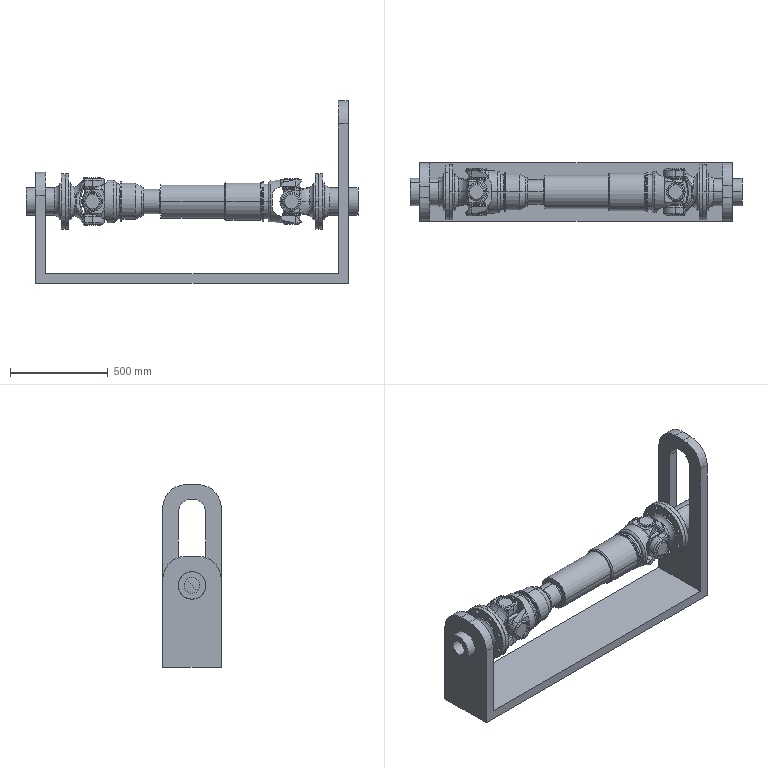Assembly | NX | mm | 10 component files | 38 solids | 702 faces | box 1700 x 300 x 936.56 mm | volume 77228193 mm3 | cylinder 314 | plane 174 | torus 122 | spline 48 | cone 36 | sphere 8 | commonest cylinder face diameters 20.1 x64 14 x56 83 x40 92 x20 90 x16 30 x8 24 x8 157.541 x8
Bill of materials:
unnamed part 1 | 2 |  | Flanged fork: a circular flat flange with a short raised hub, carrying two parallel lugs (a fork shape) that each have a round bore. The two bores share one axis.
unnamed part 2 | 1 |  | Fork attached to a stepped cylindrical shaft: a two-lug fork with coaxial round bores at one end, a larger round body with a raised ring and stepped diameters, and then a long smaller-diameter shaft.
unnamed part 3 | 1 |  | U-shaped bracket made from flat strip: a long flat base with two upright tabs at the ends that have rounded tops. One upright is taller than the other. One tab has a round hole and the other has an elongated slot.
unnamed part 4 | 1 |  | Fork attached to a cylindrical tube or shaft: a two-lug fork with coaxial round bores at one end, a short collar with a ring groove or rib, a larger cylindrical sleeve section, and then a long plain cylinder of smaller diameter.
unnamed part 5 | 1 |  | Plain solid cylinder with flat ends. Its length is about equal to its diameter.
unnamed part 6 | 2 |  | Cross-shaped body with four cylindrical arms (trunnions) sticking out from a rounded square centre block. The arms lie in one plane and are at 90° to each other.
unnamed part 7 | 2 |  | Flanged tube or spigot: a circular flat flange with eight bolt holes, and a cylindrical body sticking out from one side with a curved fillet transition. The flange face has a large central recess shaped like a bowl or counterbore.
Mates:
1. fix | model82 1 component
2. distance | model82 1 face | BRIDA2_587_Predeterminado_Como_mecanizada 1 face
3. touch align | model82 1 face | BRIDA2_587_Predeterminado_Como_mecanizada 1 face
4. touch align | BRIDA2_587_Predeterminado_Como_mecanizada 1 face | BRIDA_587_Predeterminado_Como_mecanizada 1 face
5. touch align | BRIDA_587_Predeterminado_Como_mecanizada 1 face | BRIDA2_587_Predeterminado_Como_mecanizada 1 face
6. touch align | BRIDA2_587_Predeterminado_Como_mecanizada 1 face | BRIDA_587_Predeterminado_Como_mecanizada 1 face
7. touch align | CRUZ_587_Predeterminado_Como_mecanizada 1 face | BRIDA_587_Predeterminado_Como_mecanizada 1 face
8. center | BRIDA_587_Predeterminado_Como_mecanizada 1 face | BRIDA_587_Predeterminado_Como_mecanizada 1 face | CRUZ_587_Predeterminado_Como_mecanizada 1 face | CRUZ_587_Predeterminado_Como_mecanizada 1 face
9. center | BRAZO_Predeterminado_Como_mecanizada 1 face | BRAZO_Predeterminado_Como_mecanizada 1 face | CRUZ_587_Predeterminado_Como_mecanizada 1 face | CRUZ_587_Predeterminado_Como_mecanizada 1 face
10. touch align | BRAZO_Predeterminado_Como_mecanizada 1 face | CRUZ_587_Predeterminado_Como_mecanizada 1 face
11. touch align | BRAZO_HUECO_Predeterminado_Como_mecanizada 1 face | BRAZO_Predeterminado_Como_mecanizada 1 face
12. touch align | CRUZ_587_Predeterminado_Como_mecanizada 2 face | BRAZO_HUECO_Predeterminado_Como_mecanizada 1 face
13. center | BRAZO_HUECO_Predeterminado_Como_mecanizada 1 face | BRAZO_HUECO_Predeterminado_Como_mecanizada 1 face | CRUZ_587_Predeterminado_Como_mecanizada 2 face | CRUZ_587_Predeterminado_Como_mecanizada 2 face
14. touch align | BRIDA_587_Predeterminado_Como_mecanizada 2 face | CRUZ_587_Predeterminado_Como_mecanizada 2 face
15. center | BRIDA_587_Predeterminado_Como_mecanizada 2 face | BRIDA_587_Predeterminado_Como_mecanizada 2 face | CRUZ_587_Predeterminado_Como_mecanizada 2 face | CRUZ_587_Predeterminado_Como_mecanizada 2 face
16. touch align | BRIDA2_587_Predeterminado_Como_mecanizada 2 face | BRIDA_587_Predeterminado_Como_mecanizada 2 face
17. touch align | BRIDA_587_Predeterminado_Como_mecanizada 2 face | BRIDA2_587_Predeterminado_Como_mecanizada 2 face
18. touch align | BRIDA2_587_Predeterminado_Como_mecanizada 2 face | BRIDA_587_Predeterminado_Como_mecanizada 2 face
19. parallel | CRUZ_587_Predeterminado_Como_mecanizada 1 face | model82 1 face
20. parallel | CRUZ_587_Predeterminado_Como_mecanizada 1 face | model82 1 face
21. parallel | CRUZ_587_Predeterminado_Como_mecanizada 2 face | model82 1 face
22. parallel | BRIDA2_587_Predeterminado_Como_mecanizada 2 face | model82 1 face
23. distance | BRIDA2_587_Predeterminado_Como_mecanizada 2 face | model82 1 face